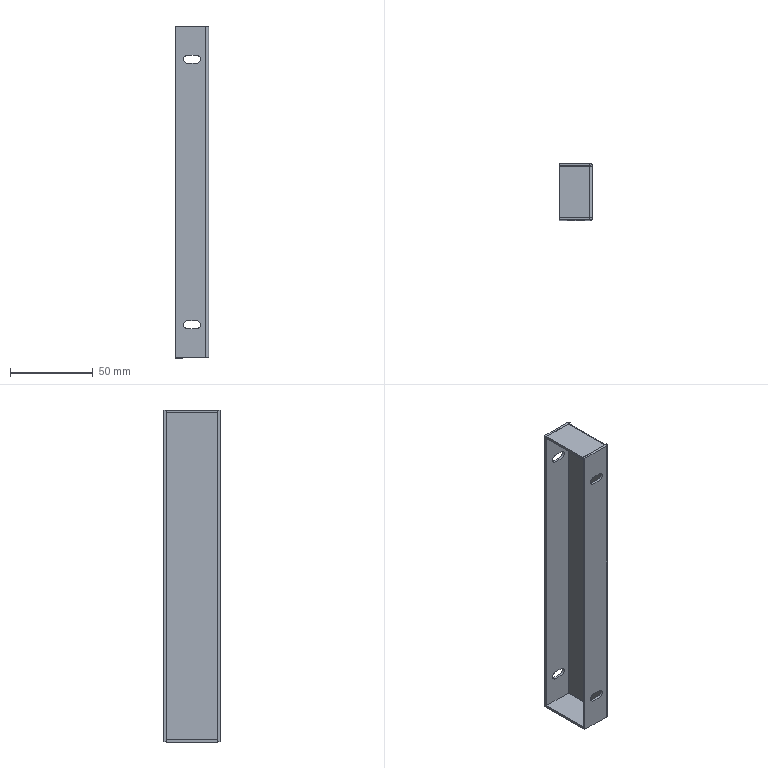Component | SolidWorks | GuideRail-1 | 1 solid | 58 faces | volume 22489 mm3 | plane 42 | cylinder 16 | commonest cylinder face diameters 5 x8 0.2 x4 3.2 x4